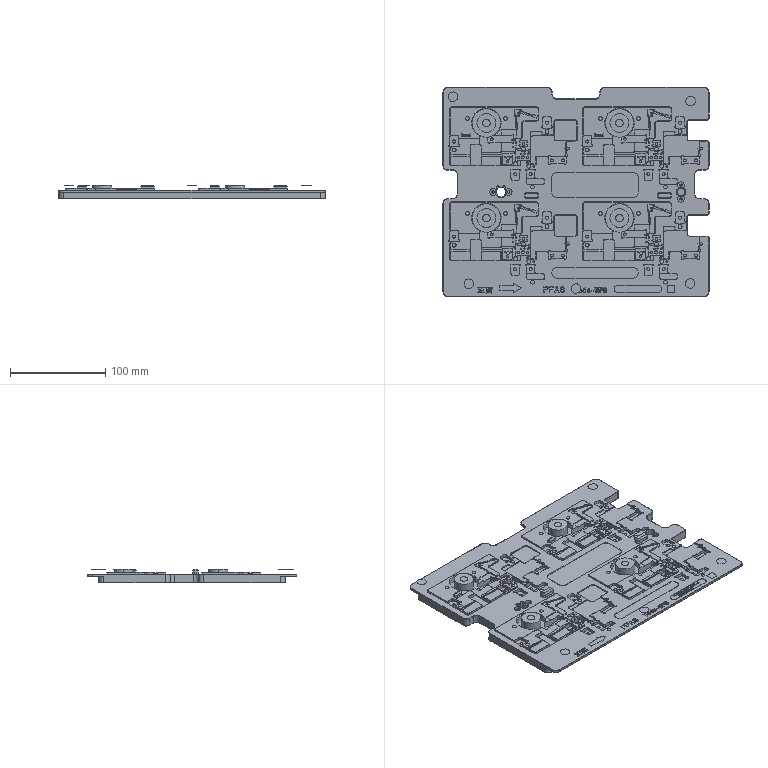CAM job | Mastercam | mm | 67 operations | part box 285 x 225 x 14.7
1. Facing | 1 - 80 面铣
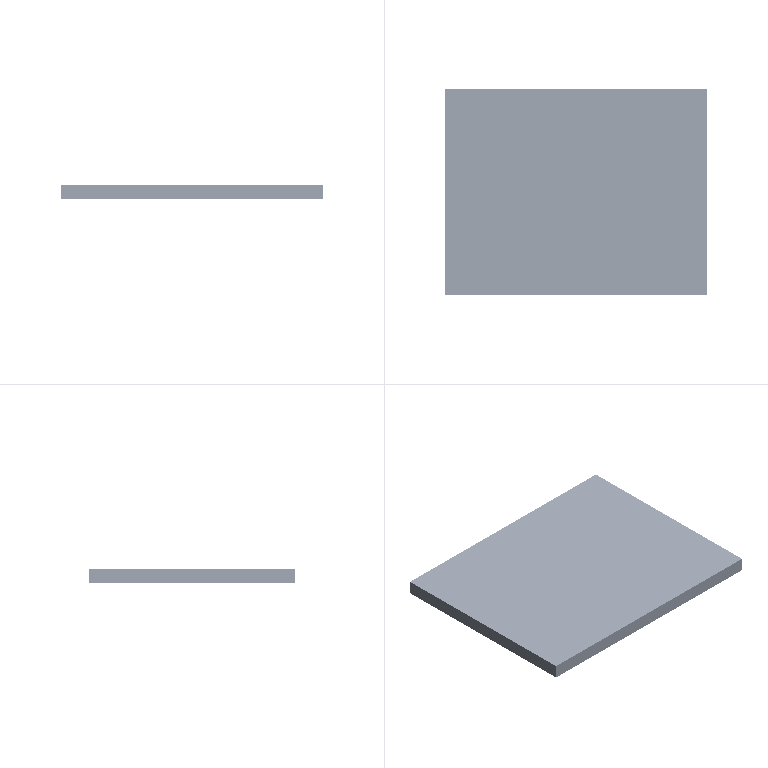2. Surface Rough Pocket | 9 - 10C 平底刀
3. Drill/Counterbore | 2 - 6定位倒角
4. Peck Drill | 18 - 4.5 钻头
5. Helix Bore | 7 - 4 平底刀
6. 3D High Speed (Area rest roughing) | 6 - 6 平底刀
7. Facing | 1 - 80 面铣
8. Contour (Ramp) | 9 - 10C 平底刀
9. Facing | 9 - 10C 平底刀
10. Contour (2D) | 9 - 10C 平底刀
11. Contour (Ramp) | 7 - 4 平底刀
12. Drill/Counterbore | 2 - 4定位倒角
13. Peck Drill | 17 - 1 钻头
14. Peck Drill | 19 - 1.3 钻头
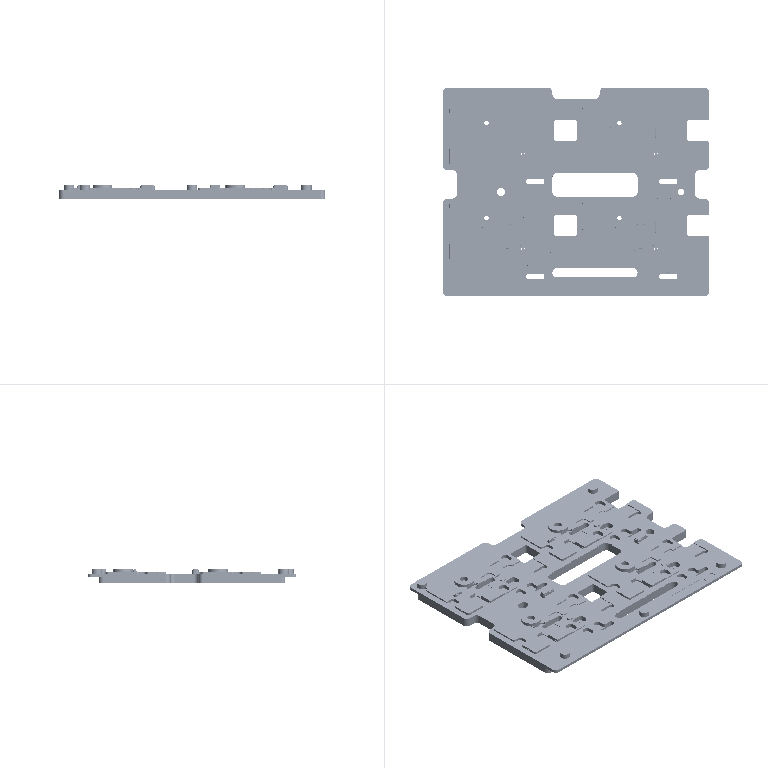15. Peck Drill | 20 - 1.5 钻头
16. Peck Drill | 11 - 1.6 钻头
17. Peck Drill | 11 - 1.6 钻头
18. Peck Drill | 15 - 1.7 钻头
19. Peck Drill | 12 - 2 钻头
20. Peck Drill | 21 - 2.5 钻头
21. Peck Drill | 14 - 2.7 钻头
22. Peck Drill | 13 - 3 钻头
23. Peck Drill | 16 - 3.2 钻头
24. Pocket (Standard) | 4 - 2 平铣刀
25. Contour (Remachining) | 24 - 1 平铣刀
26. Contour (2D) | 4 - 2 平铣刀
27. Helix Bore | 3 - 3 平铣刀
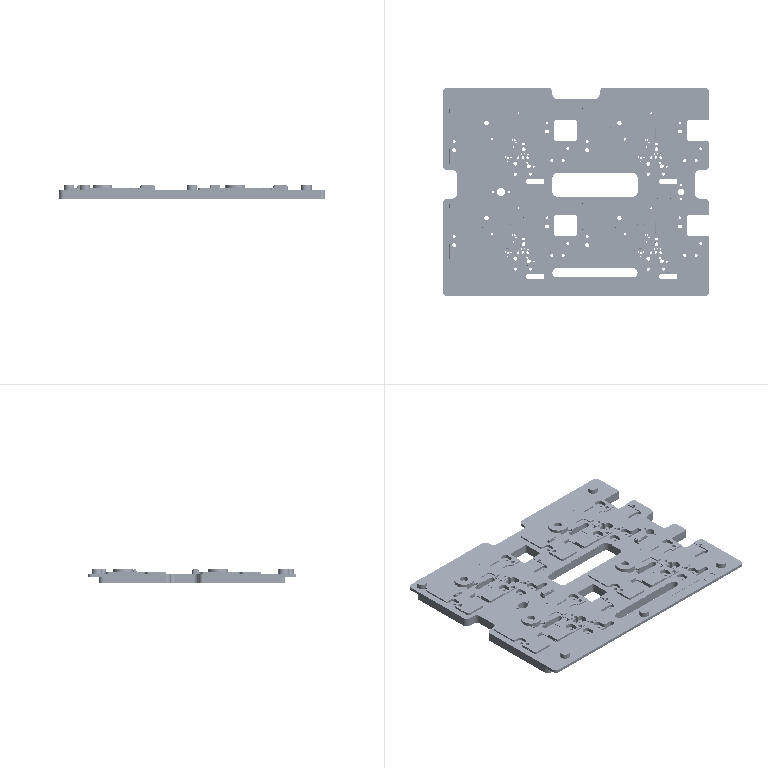28. Helix Bore | 3 - 3 平铣刀
29. Helix Bore | 24 - 1 平铣刀
30. Helix Bore | 5 - 1.5 平铣刀
31. Helix Bore | 5 - 1.5 平铣刀
32. Helix Bore | 4 - 2 平铣刀
33. Helix Bore | 3 - 3 平铣刀
34. Helix Bore | 3 - 3 平铣刀
35. Helix Bore | 7 - 4 平底刀
36. Helix Bore | 6 - 6 平底刀
37. Contour (2D) | 10 - 10J 平底刀
38. Contour (2D) | 8 - 4 J平底刀
39. Model Chamfer | 2 - 4定位倒角
40. Model Chamfer | 2 - 4定位倒角
41. Facing | 10 - 10J 平底刀
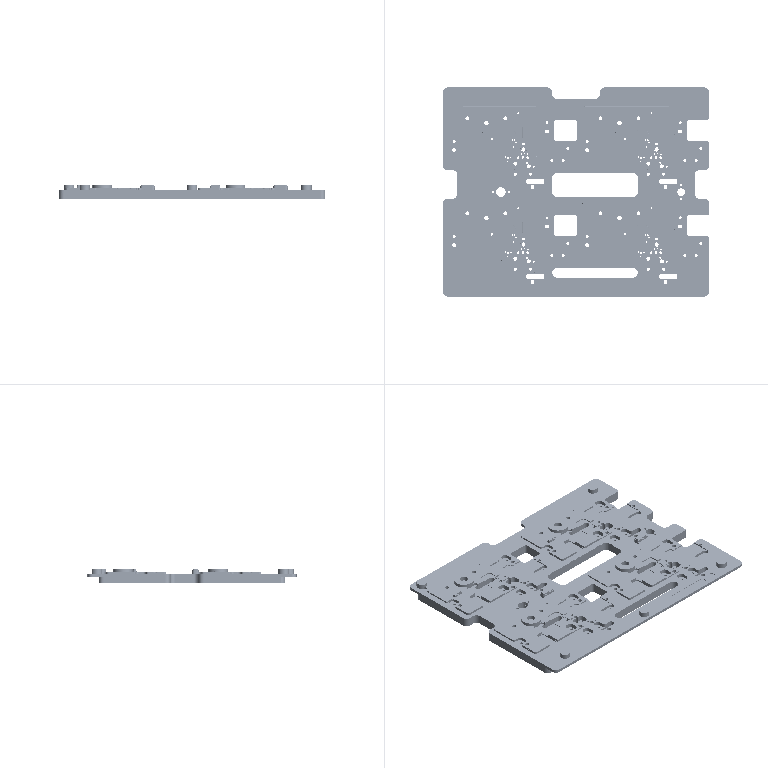42. Unified Morph 5axis OP | 23 - 4 -R0.5圆鼻铣刀
43. Unified Morph 5axis OP | 23 - 4 -R0.5圆鼻铣刀
44. Facing | 5 - 8 平底刀
45. Facing | 5 - 8 平底刀
46. 3D High Speed (Area rest roughing) | 5 - 8 平底刀
47. 挖槽清角策略 | 7 - 4 平底刀
48. 挖槽清角策略 | 3 - 3 平铣刀
49. Surface Rough Pocket | 8 - 4 J平底刀
50. 3D High Speed (Waterline) | 8 - 4 J平底刀
51. 挖槽清角策略 | 4 - 2 平铣刀
52. 挖槽清角策略 | 24 - 1 平铣刀
53. 3D High Speed (Waterline) | 24 - 1 平铣刀
54. Contour (Remachining) | 22 - 0.8 平铣刀
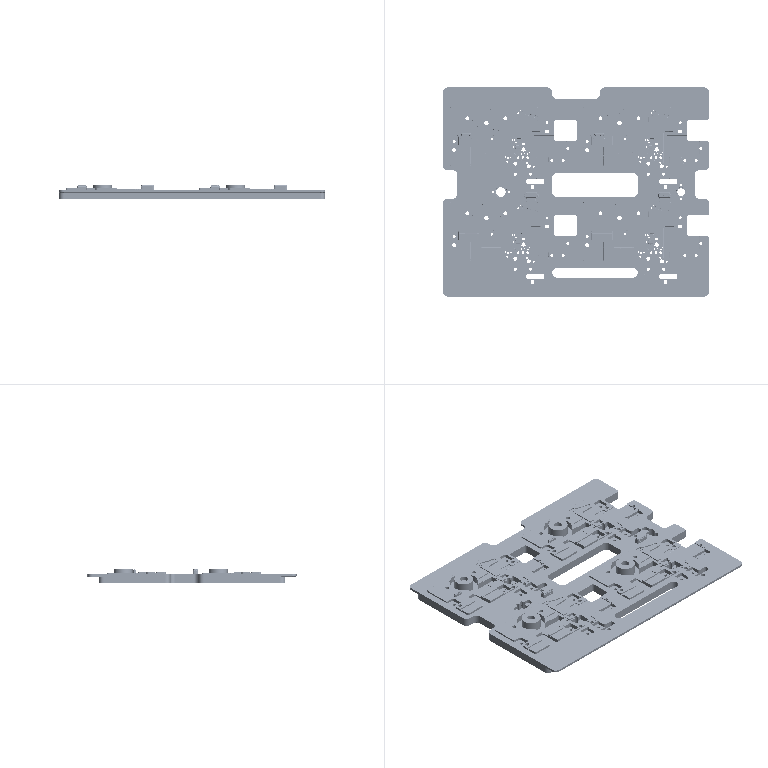55. Contour (2D) | 3 - 3 平铣刀
56. Pocket (Standard) | 4 - 2 平铣刀
57. Contour (Remachining) | 24 - 1 平铣刀
58. Model Chamfer | 2 - 4定位倒角
59. Model Chamfer | 2 - 4定位倒角
60. Unified Morph 5axis OP | 23 - 4 -R0.5圆鼻铣刀
61. Unified Morph 5axis OP | 23 - 4 -R0.5圆鼻铣刀
62. 3D High Speed (Raster) | 23 - 4 -R0.5圆鼻铣刀
63. Circle Mill | 6 - 6 平底刀
64. Contour (2D) | 4 - 2 平铣刀
65. Contour (2D) | 6 - 6 平底刀
66. Contour (Ramp) | 9 - 10C 平底刀
67. Contour (2D) | 5 - 8 J平底刀